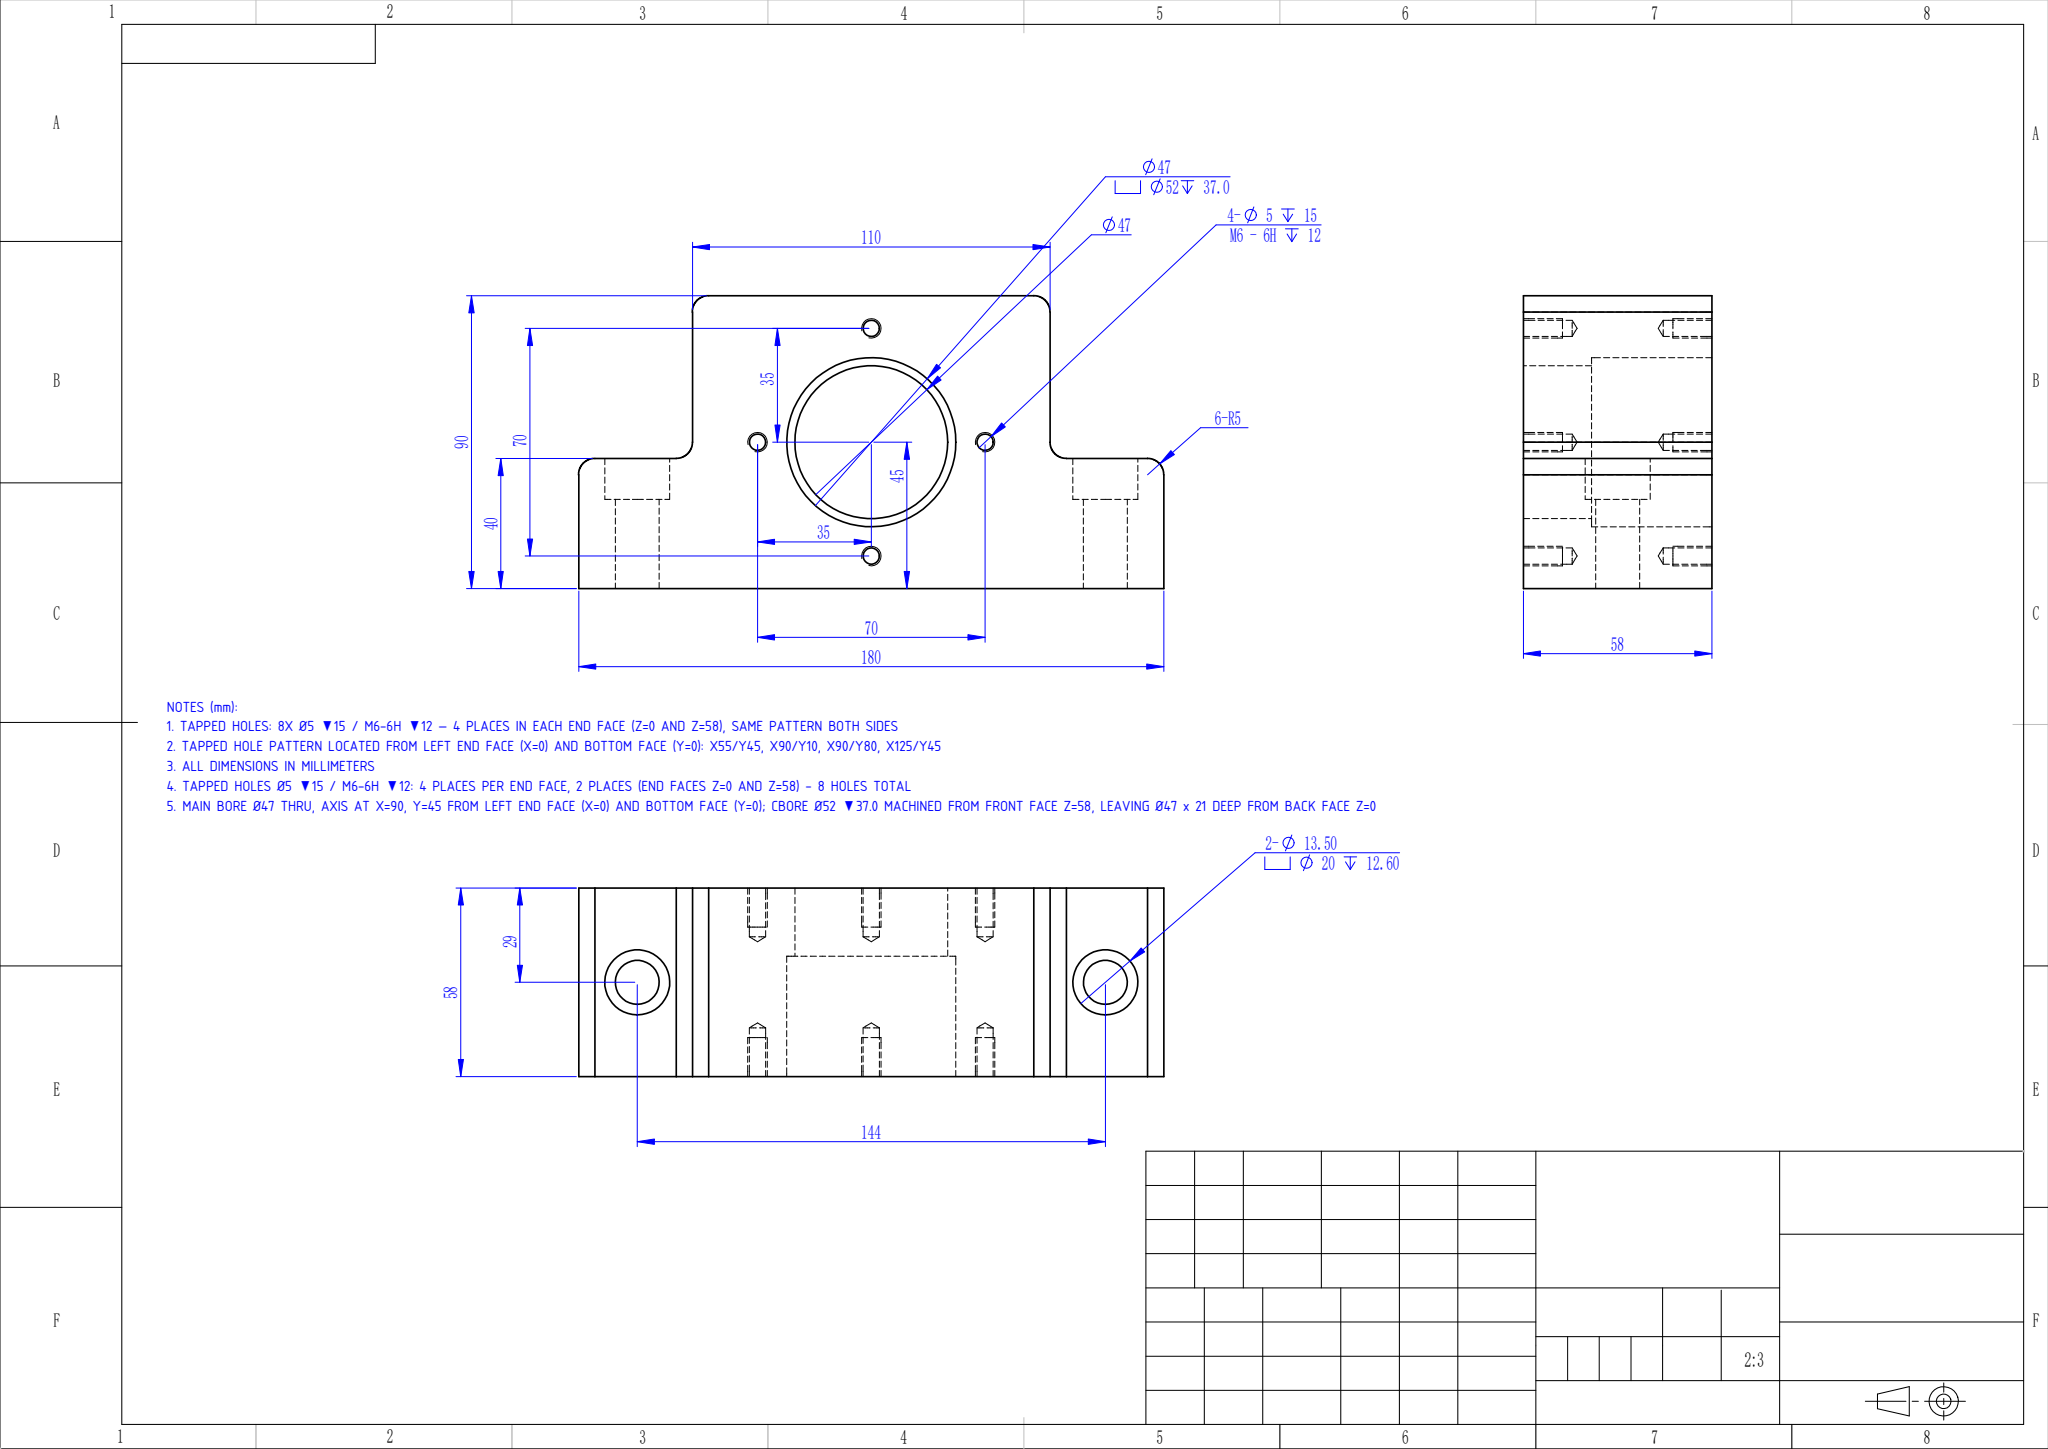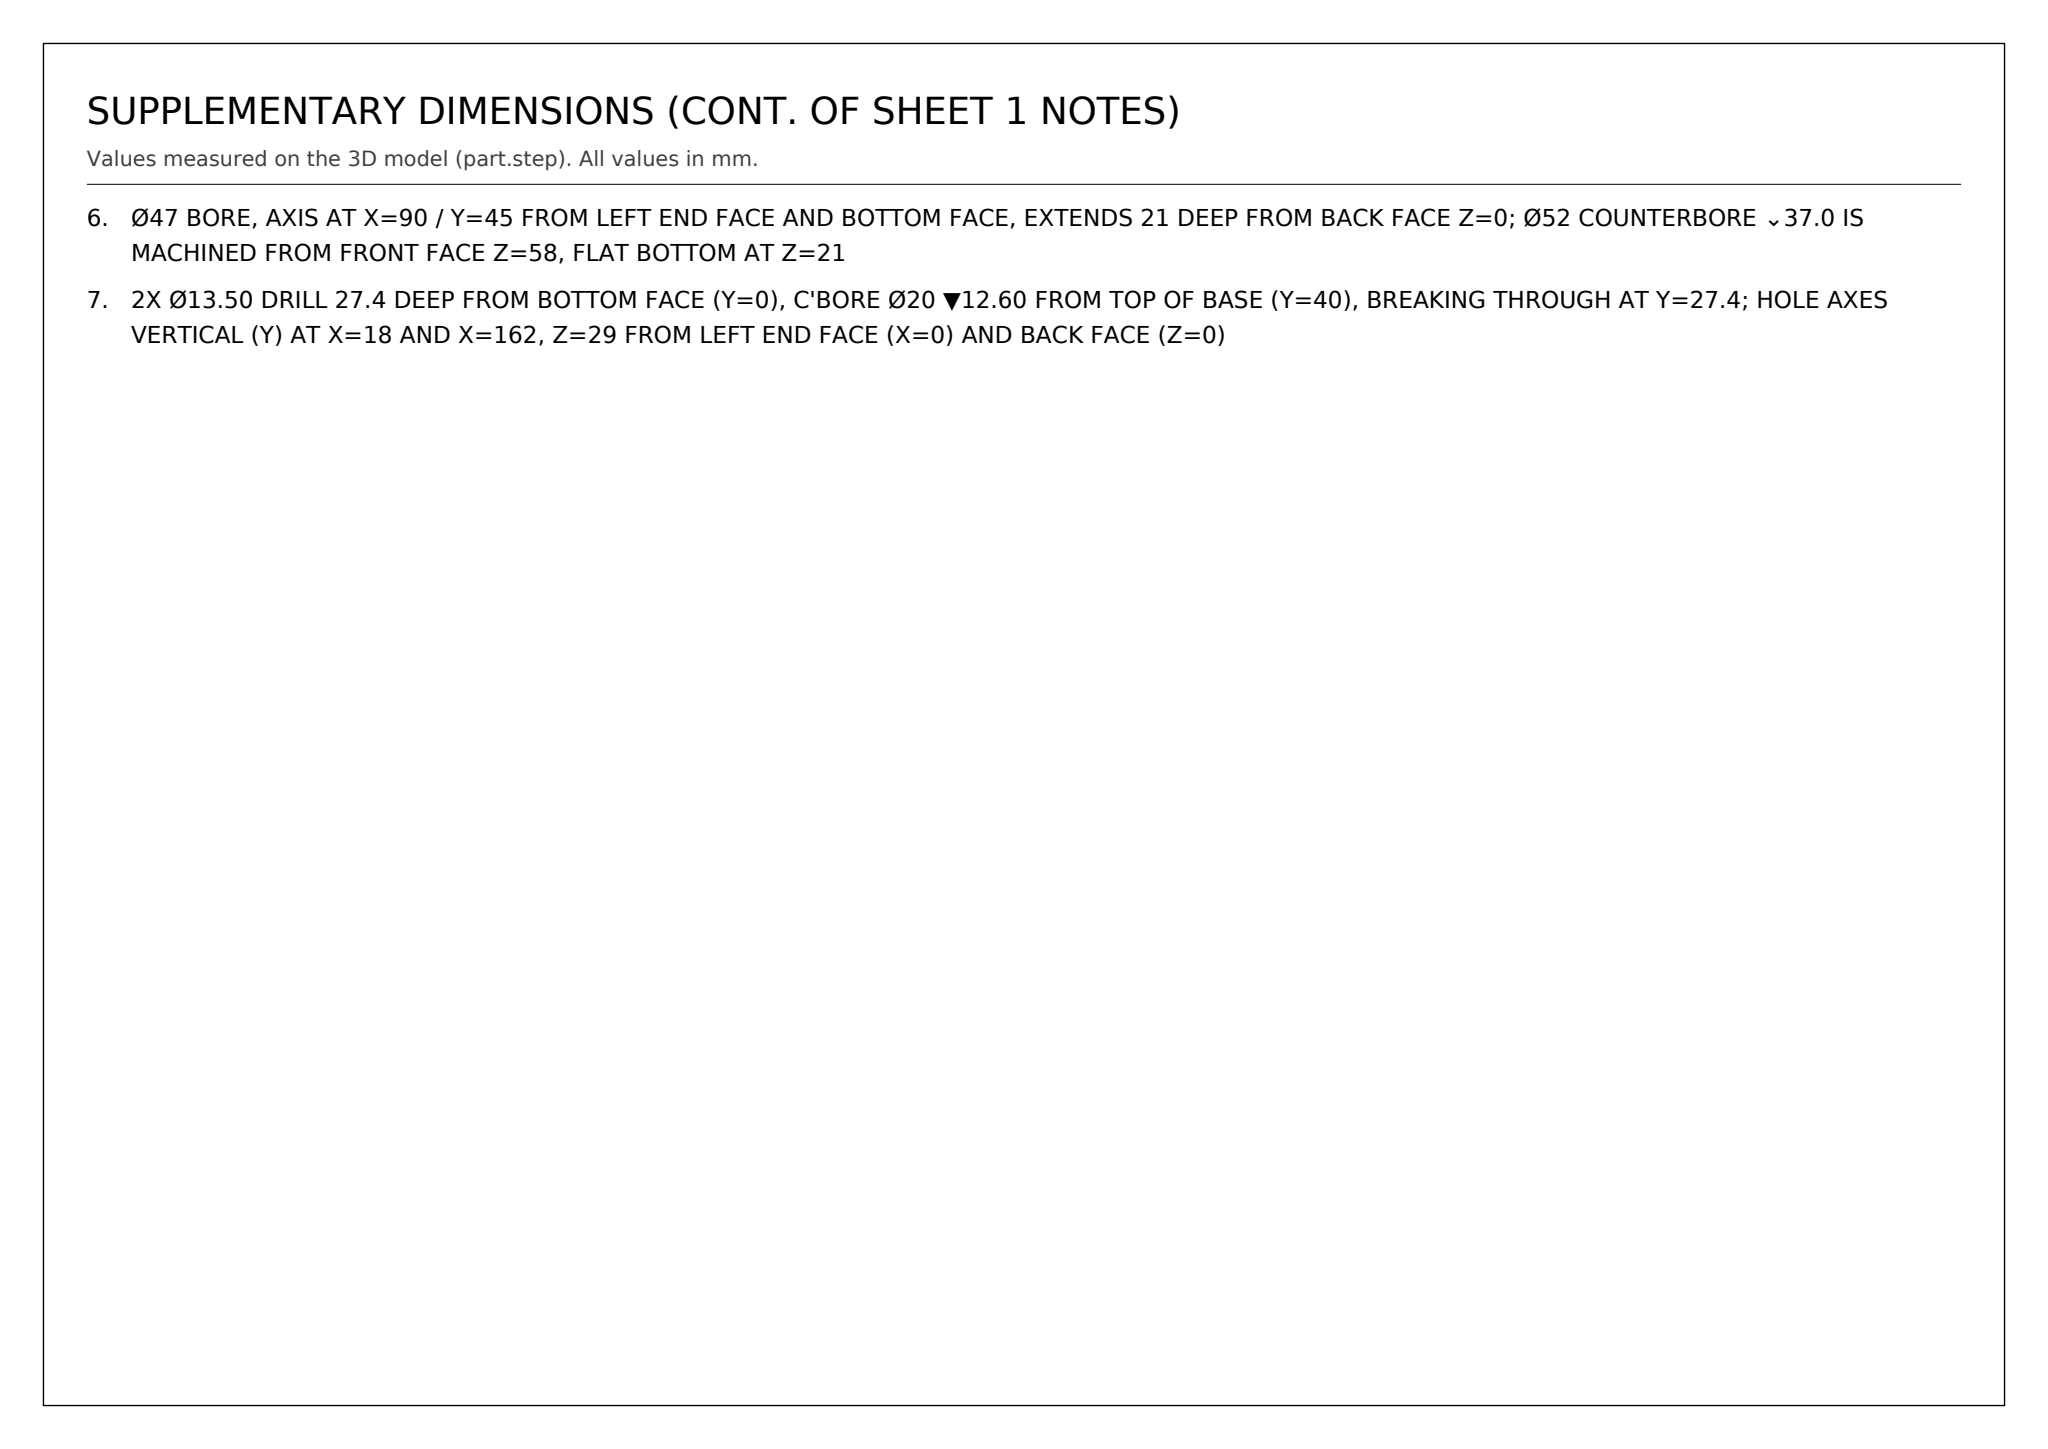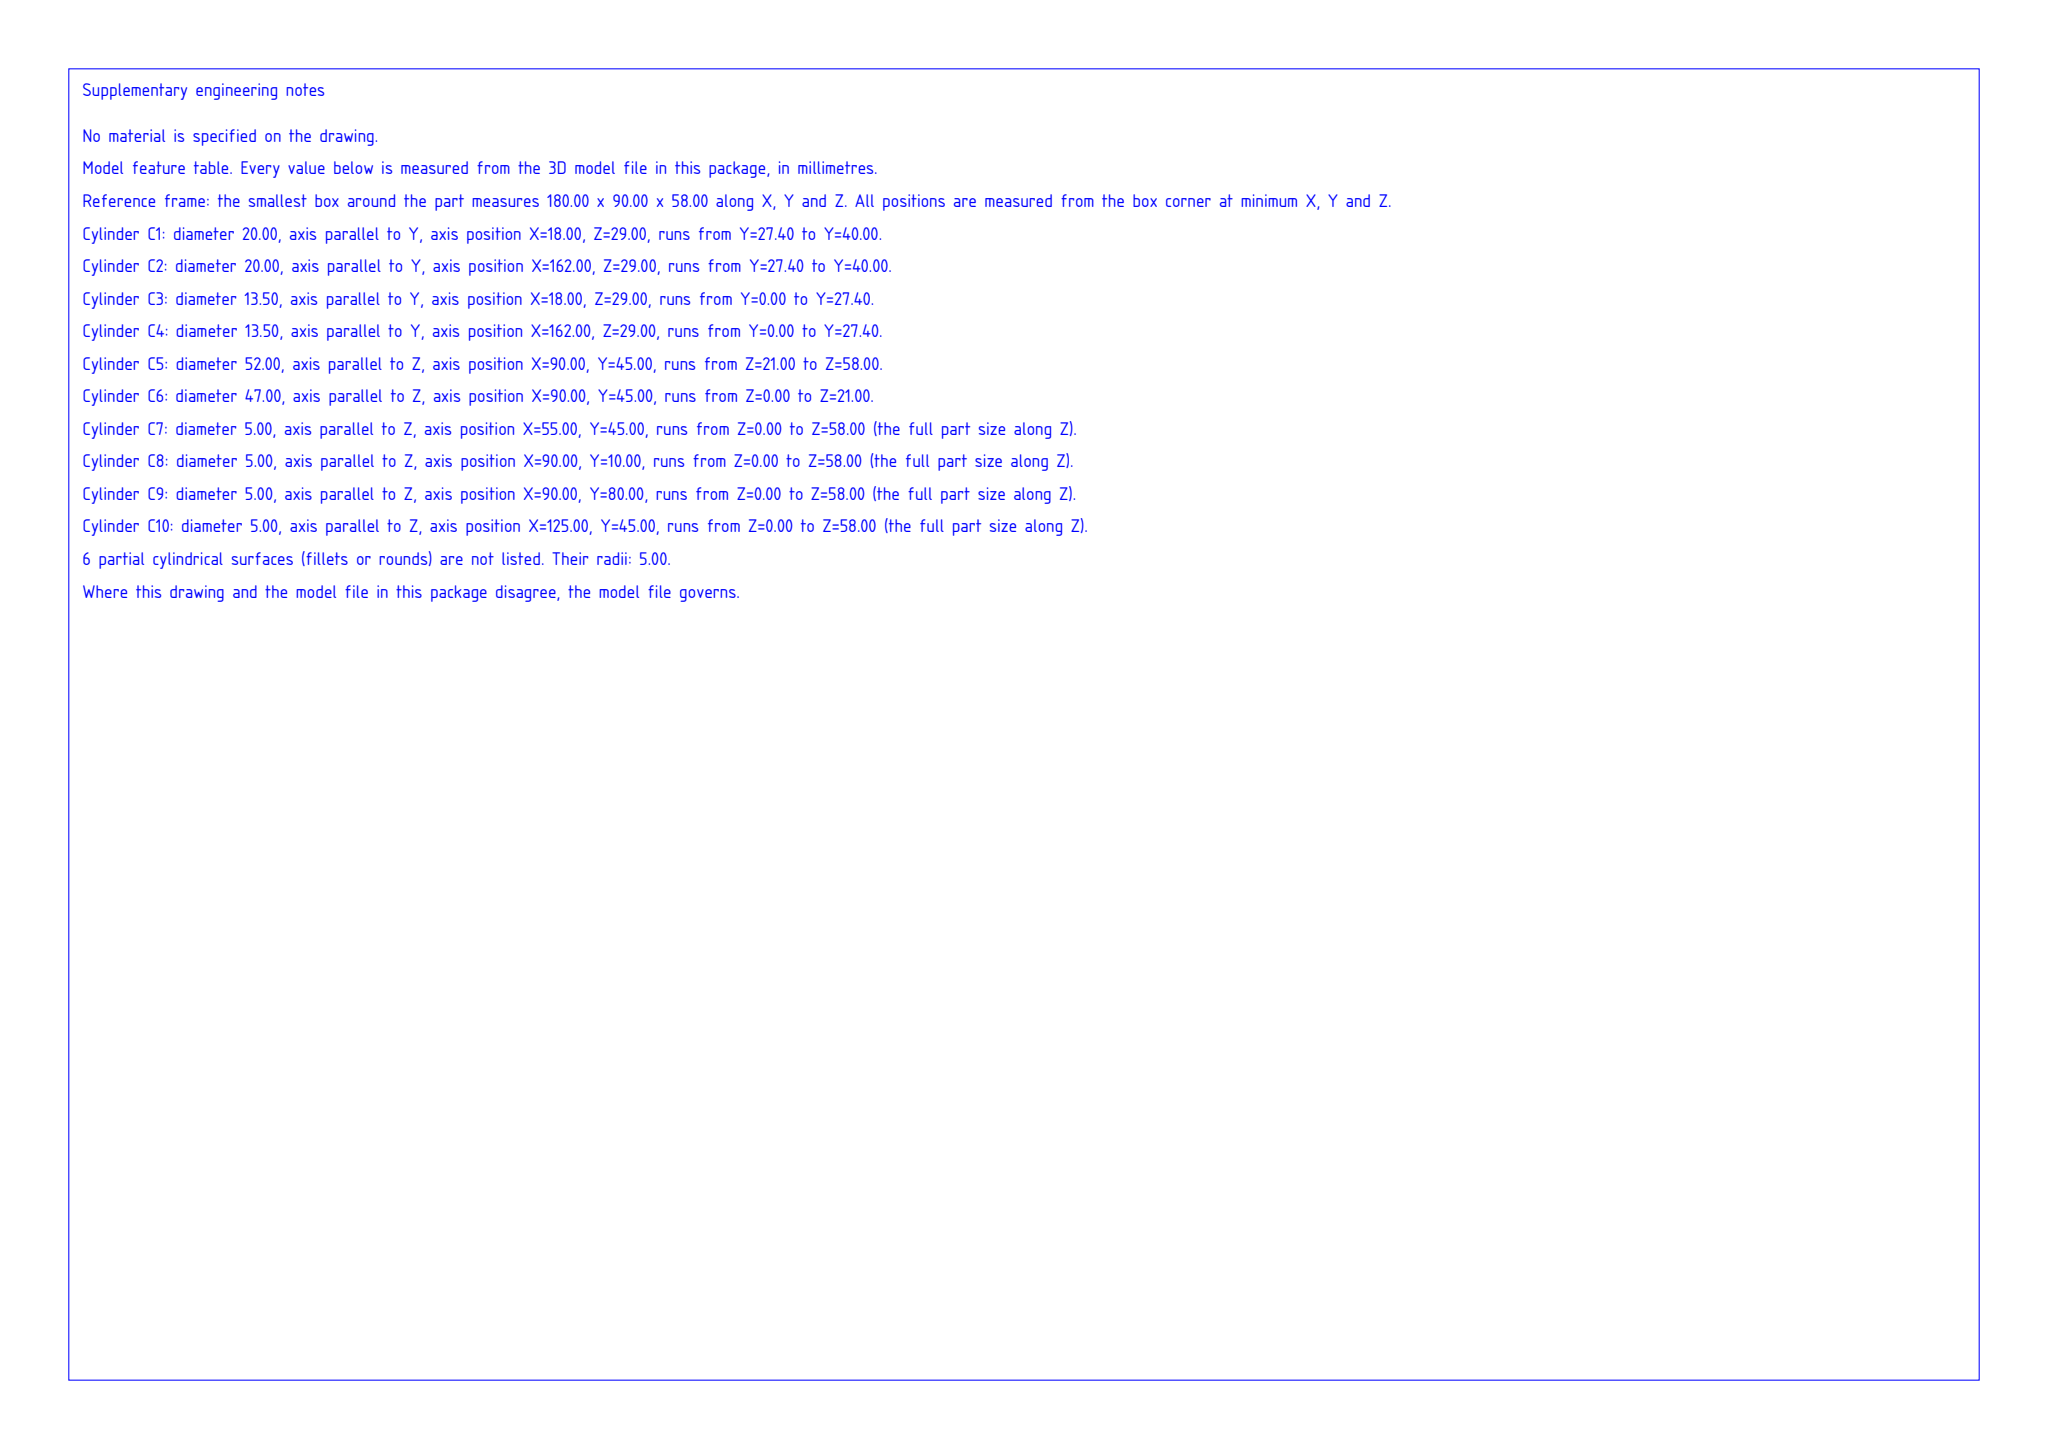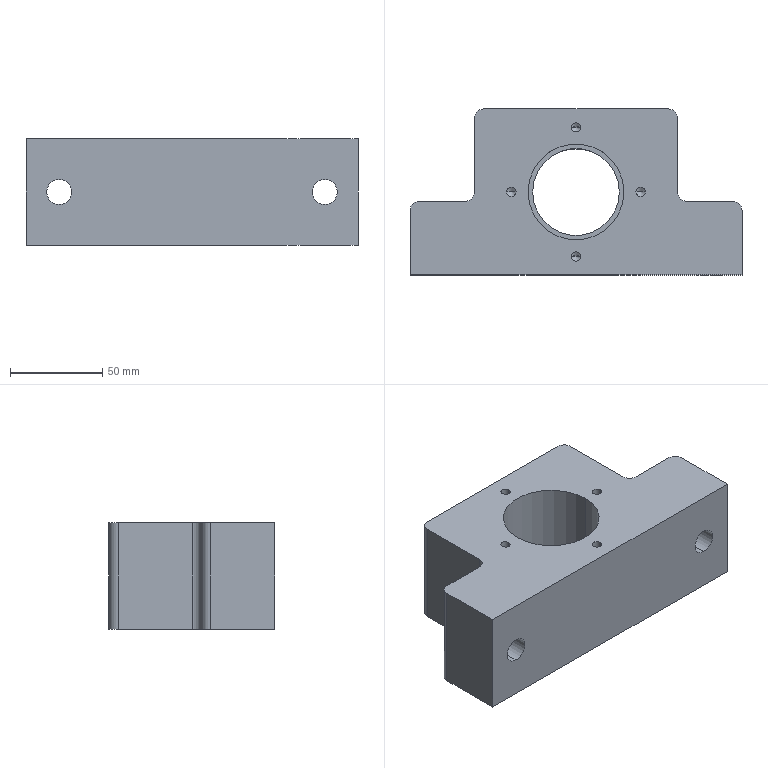Part | SolidWorks | mm | 1 solid | 63 faces | box 180 x 90 x 58 mm | volume 602771 mm3 | cylinder 34 | cone 16 | plane 13 | commonest cylinder face diameters 5 x16 10 x6 20 x4 13.5 x4 52 x2 47 x2
Drawing notes:
TAPPED HOLES: 8X Ø5 ▼15 / M6-6H ▼12 — 4 PLACES IN EACH END FACE (Z=0 AND Z=58), SAME PATTERN BOTH SIDES | from the solid: cylinders dia 5.0 axis z length 15.0 at (55,45), (90,10), (90,80), (125,45); z-planes at 0.0 and 58.0 with cones 118° ref dia 5.0 (16 drill points = 8 holes x 2 ends)
TAPPED HOLE PATTERN LOCATED FROM LEFT END FACE (X=0) AND BOTTOM FACE (Y=0): X55/Y45, X90/Y10, X90/Y80, X125/Y45 | from the solid: cylinders dia 5.0 pos_other_axes [55,45], [90,10], [90,80], [125,45] from min corner of bbox
ALL DIMENSIONS IN MILLIMETERS | from the solid: STEP model units mm; bbox_xyz 180.0 x 90.0 x 58.0
TAPPED HOLES Ø5 ▼15 / M6-6H ▼12: 4 PLACES PER END FACE, 2 PLACES (END FACES Z=0 AND Z=58) - 8 HOLES TOTAL | from the solid: cylinders dia 5.0 axis z length 15 at XY 55/45, 90/10, 90/80, 125/45 with bbox_z=58 (holes from both Z=0 and Z=58 faces); cones 118deg ref_dia 5.0 count 16
MAIN BORE Ø47 THRU, AXIS AT X=90, Y=45 FROM LEFT END FACE (X=0) AND BOTTOM FACE (Y=0); CBORE Ø52 ▼37.0 MACHINED FROM FRONT FACE Z=58, LEAVING Ø47 x 21 DEEP FROM BACK FACE Z=0 | from the solid: cylinders: [47.0,'z',[90,45],21.0] and [52.0,'z',[90,45],37.0]; axis_planes z=0, z=21, z=58; bbox_xyz Z=58
Ø47 BORE, AXIS AT X=90 / Y=45 FROM LEFT END FACE AND BOTTOM FACE, EXTENDS 21 DEEP FROM BACK FACE Z=0; Ø52 COUNTERBORE ⌄37.0 IS MACHINED FROM FRONT FACE Z=58, FLAT BOTTOM AT Z=21 | from the solid: cylinders [47.0,'z',[90,45],21.0] and [52.0,'z',[90,45],37.0]; axis_planes z=0, z=21, z=58 with bbox_xyz Z=58
2X Ø13.50 DRILL 27.4 DEEP FROM BOTTOM FACE (Y=0), C'BORE Ø20 ▼12.60 FROM TOP OF BASE (Y=40), BREAKING THROUGH AT Y=27.4; HOLE AXES VERTICAL (Y) AT X=18 AND X=162, Z=29 FROM LEFT END FACE (X=0) AND BACK FACE (Z=0) | from the solid: cylinders [13.5,"y",[18.0,null,29.0],27.4,2] and [13.5,"y",[162.0,null,29.0],27.4,2]; [20.0,"y",[18.0,null,29.0],12.6,2] and [20.0,"y",[162.0,null,29.0],12.6,2]; axis_planes y=0.0, y=27.4, y=40.0
build123d program:
from build123d import *

# Parameters (mm, degrees)
SKETCH1_R                                        = 23.5
BOSS_EXTRUDE1_DEPTH                              = 58
M12_HEX_SOCKET_HEAD_CAP_SCREW_CBORE1_D           = 13.5
M12_HEX_SOCKET_HEAD_CAP_SCREW_CBORE1_CBORE_D     = 20
M12_HEX_SOCKET_HEAD_CAP_SCREW_CBORE1_CBORE_DEPTH = 12.6
FILLET1_R                                        = 5
CIRPATTERN1_COUNT                                = 4
SKETCH9_R                                        = 26
CUT_EXTRUDE1_DEPTH                               = 37


with BuildPart() as part:
    # Sketch1 → Boss-Extrude1 (new body)
    with BuildSketch(Plane.XY):
        Polygon((55, 0), (-55, 0), (-55, -50), (-90, -50), (-90, -90), (90, -90), (90, -50), (55, -50), align=None)
        with Locations((0, -45)):
            Circle(SKETCH1_R, mode=Mode.SUBTRACT)
    extrude(amount=-BOSS_EXTRUDE1_DEPTH)

    # Sketch2 → M6 Tapped Hole1 (revolve, cut)
    with BuildSketch(Plane(origin=(0, -10, 0), x_dir=(0, -1, 0), z_dir=(1, 0, 0))):
        Polygon((0, 0), (0, 16.502), (2.5, 15), (2.5, 0), align=None)
    m6_tapped_hole1 = revolve(axis=Axis((0, -10, 6.35), (0, 0, -1)), mode=Mode.SUBTRACT)

    # M12 Hex Socket Head Cap Screw CBORE1 (through all)
    with Locations(Plane(origin=(0, -50, 0), x_dir=(1, 0, 0), z_dir=(0, 1, 0))):
        with Locations((-72, 29)):
            m12_hex_socket_head_cap_screw_cbore1 = CounterBoreHole(M12_HEX_SOCKET_HEAD_CAP_SCREW_CBORE1_D / 2, M12_HEX_SOCKET_HEAD_CAP_SCREW_CBORE1_CBORE_D / 2, M12_HEX_SOCKET_HEAD_CAP_SCREW_CBORE1_CBORE_DEPTH)

    # Mirror4: M12 Hex Socket Head Cap Screw CBORE1 across plane
    add(m12_hex_socket_head_cap_screw_cbore1.mirror(Plane(origin=(0, 0, 0), x_dir=(0, 0, 1), z_dir=(1, 0, 0))), mode=Mode.SUBTRACT)

    # Fillet1
    fillet1_edges = [part.edges().sort_by_distance(p)[0] for p in [
        (-55, 0, -29),
        (55, 0, -29),
        (55, -50, -29),
        (90, -50, -29),
        (-90, -50, -29),
        (-55, -50, -29),
    ]]
    fillet(fillet1_edges, radius=FILLET1_R)

    # CirPattern1: M6 Tapped Hole1 ×4 about axis
    cirpattern1_axis = Axis((0, -45, 0), (0, 0, 1))
    for i in range(1, CIRPATTERN1_COUNT):
        add(m6_tapped_hole1.rotate(cirpattern1_axis, i * 360 / CIRPATTERN1_COUNT), mode=Mode.SUBTRACT)

    # Mirror5: M6 Tapped Hole1 across plane
    add(m6_tapped_hole1.mirror(Plane.XY.offset(-29)), mode=Mode.SUBTRACT)

    # Mirror5 copy 1 sketch → Mirror5 copy 1 (revolve, cut)
    with BuildSketch(Plane(origin=(-35, -45, -58), x_dir=(1, 0, 0), z_dir=(0, 1, 0))):
        Polygon((0, 0), (0, -16.502), (2.5, -15), (2.5, 0), align=None)
    revolve(axis=Axis((-35, -45, -64.35), (0, 0, -1)), mode=Mode.SUBTRACT)

    # Mirror5 copy 2 sketch → Mirror5 copy 2 (revolve, cut)
    with BuildSketch(Plane(origin=(0, -80, -58), x_dir=(0, 1, 0), z_dir=(-1, 0, 0))):
        Polygon((0, 0), (0, -16.502), (2.5, -15), (2.5, 0), align=None)
    revolve(axis=Axis((0, -80, -64.35), (0, 0, -1)), mode=Mode.SUBTRACT)

    # Mirror5 copy 3 sketch → Mirror5 copy 3 (revolve, cut)
    with BuildSketch(Plane(origin=(35, -45, -58), x_dir=(-1, 0, 0), z_dir=(0, -1, 0))):
        Polygon((0, 0), (0, -16.502), (2.5, -15), (2.5, 0), align=None)
    revolve(axis=Axis((35, -45, -64.35), (0, 0, -1)), mode=Mode.SUBTRACT)

    # Sketch9 → Cut-Extrude1 (cut)
    with BuildSketch(Plane.XY):
        with Locations((0, -45)):
            Circle(SKETCH9_R)
    extrude(amount=-CUT_EXTRUDE1_DEPTH, mode=Mode.SUBTRACT)


solid = part.part